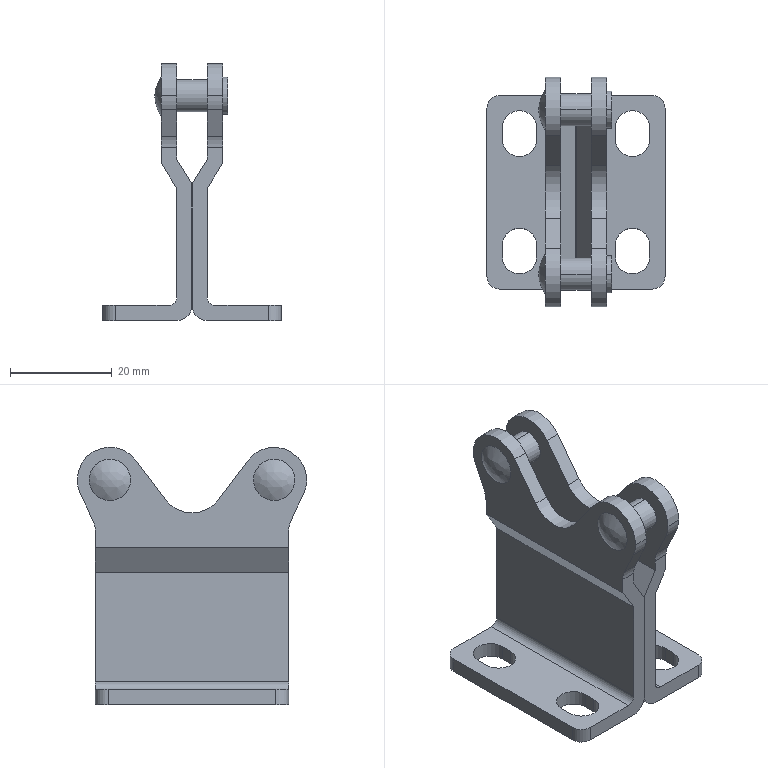Component | SolidWorks | AD12-MC01H-4_2_03.SDASM-1_AD12-_MC01H-4_bod.sdprt-1 | 1 solid | 82 faces | volume 13968 mm3 | plane 44 | cylinder 36 | spline 2 | commonest cylinder face diameters 6.7 x8 12.8 x6 6.35 x4 7.35 x4 5 x4 10 x4 3 x2 6 x2